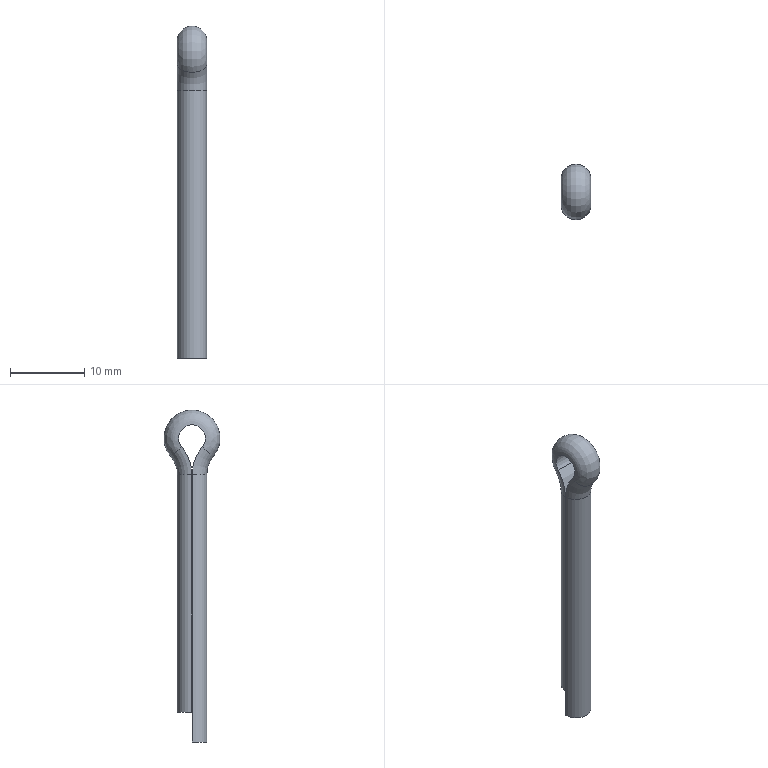Component | NX | 3_COTTER_PIN | 1 solid | 12 faces | box 4 x 7.55 x 44.7 mm | volume 545 mm3 | cylinder 5 | plane 4 | torus 2 | spline 1 | commonest cylinder face diameters 4 x2 11.596 x2 3.596 x1
STEP:
#1=VALUE_REPRESENTATION_ITEM('',COUNT_MEASURE(0.));
#2=(LENGTH_UNIT()NAMED_UNIT(*)SI_UNIT(.MILLI.,.METRE.));
#3=UNCERTAINTY_MEASURE_WITH_UNIT(LENGTH_MEASURE(0.0254),#2,'','');
#4=(NAMED_UNIT(*)PLANE_ANGLE_UNIT()SI_UNIT($,.RADIAN.));
#5=PLANE_ANGLE_MEASURE_WITH_UNIT(PLANE_ANGLE_MEASURE(0.01745),#4);
#6=DIMENSIONAL_EXPONENTS(0.,0.,0.,0.,0.,0.,0.);
#7=(CONVERSION_BASED_UNIT('',#5)NAMED_UNIT(#6)PLANE_ANGLE_UNIT());
#8=(NAMED_UNIT(*)SI_UNIT($,.STERADIAN.)SOLID_ANGLE_UNIT());
#9=(GEOMETRIC_REPRESENTATION_CONTEXT(3)GLOBAL_UNCERTAINTY_ASSIGNED_CONTEXT((#3))GLOBAL_UNIT_ASSIGNED_CONTEXT((#2,#7,#8))REPRESENTATION_CONTEXT('',''));
#10=REPRESENTATION('',(#1),#9);
#11=VALUE_REPRESENTATION_ITEM('',COUNT_MEASURE(0.));
#12=REPRESENTATION('',(#11),#9);
#13=CARTESIAN_POINT('',(0.,0.,0.));
#14=DIRECTION('',(0.,0.,1.));
#15=DIRECTION('',(1.,0.,0.));
#16=AXIS2_PLACEMENT_3D('',#13,#14,#15);
#17=SHAPE_REPRESENTATION('',(#16),#9);
#18=CARTESIAN_POINT('',(36.,-0.005,112.5));
#19=VERTEX_POINT('',#18);
#20=CARTESIAN_POINT('',(40.,-0.005,112.5));
#21=VERTEX_POINT('',#20);
#22=CARTESIAN_POINT('',(36.,-0.005,112.5));
#23=DIRECTION('',(1.,0.,0.));
#24=VECTOR('',#23,1.);
#25=LINE('',#22,#24);
#26=EDGE_CURVE('',#19,#21,#25,.T.);
#27=ORIENTED_EDGE('',*,*,#26,.T.);
#28=CARTESIAN_POINT('',(40.,-0.005,76.5));
#29=VERTEX_POINT('',#28);
#30=CARTESIAN_POINT('',(40.,-0.005,112.5));
#31=DIRECTION('',(0.,0.,-1.));
#32=VECTOR('',#31,1.);
#33=LINE('',#30,#32);
#34=EDGE_CURVE('',#21,#29,#33,.T.);
#35=ORIENTED_EDGE('',*,*,#34,.T.);
#36=CARTESIAN_POINT('',(36.,-0.005,76.5));
#37=VERTEX_POINT('',#36);
#38=CARTESIAN_POINT('',(36.,-0.005,76.5));
#39=DIRECTION('',(1.,0.,0.));
#40=VECTOR('',#39,1.);
#41=LINE('',#38,#40);
#42=EDGE_CURVE('',#37,#29,#41,.T.);
#43=ORIENTED_EDGE('',*,*,#42,.F.);
#44=CARTESIAN_POINT('',(36.,-0.005,112.5));
#45=DIRECTION('',(0.,0.,-1.));
#46=VECTOR('',#45,1.);
#47=LINE('',#44,#46);
#48=EDGE_CURVE('',#19,#37,#47,.T.);
#49=ORIENTED_EDGE('',*,*,#48,.F.);
#50=EDGE_LOOP('',(#27,#35,#43,#49));
#51=FACE_OUTER_BOUND('',#50,.T.);
#52=CARTESIAN_POINT('',(36.,-0.005,112.5));
#53=DIRECTION('',(0.,1.,0.));
#54=DIRECTION('',(0.,0.,1.));
#55=AXIS2_PLACEMENT_3D('',#52,#53,#54);
#56=PLANE('',#55);
#57=ADVANCED_FACE('',(#51),#56,.T.);
#58=CARTESIAN_POINT('',(38.,0.,112.5));
#59=DIRECTION('',(0.,-0.,-1.));
#60=DIRECTION('',(1.,0.,0.));
#61=AXIS2_PLACEMENT_3D('',#58,#59,#60);
#62=CIRCLE('',#61,2.);
#63=EDGE_CURVE('',#21,#19,#62,.T.);
#64=ORIENTED_EDGE('',*,*,#63,.T.);
#65=ORIENTED_EDGE('',*,*,#48,.T.);
#66=CARTESIAN_POINT('',(38.,0.,76.5));
#67=DIRECTION('',(0.,-0.,-1.));
#68=DIRECTION('',(1.,0.,0.));
#69=AXIS2_PLACEMENT_3D('',#66,#67,#68);
#70=CIRCLE('',#69,2.);
#71=EDGE_CURVE('',#29,#37,#70,.T.);
#72=ORIENTED_EDGE('',*,*,#71,.F.);
#73=ORIENTED_EDGE('',*,*,#34,.F.);
#74=EDGE_LOOP('',(#64,#65,#72,#73));
#75=FACE_OUTER_BOUND('',#74,.T.);
#76=CARTESIAN_POINT('',(38.,0.,112.5));
#77=DIRECTION('',(0.,0.,-1.));
#78=DIRECTION('',(-1.,0.,0.));
#79=AXIS2_PLACEMENT_3D('',#76,#77,#78);
#80=CYLINDRICAL_SURFACE('',#79,2.);
#81=ADVANCED_FACE('',(#75),#80,.T.);
#82=CARTESIAN_POINT('',(36.,-1.374,116.241));
#83=VERTEX_POINT('',#82);
#84=CARTESIAN_POINT('',(40.,-1.374,116.241));
#85=VERTEX_POINT('',#84);
#86=CARTESIAN_POINT('',(36.,-1.374,116.241));
#87=DIRECTION('',(1.,0.,0.));
#88=VECTOR('',#87,1.);
#89=LINE('',#86,#88);
#90=EDGE_CURVE('',#83,#85,#89,.T.);
#91=ORIENTED_EDGE('',*,*,#90,.T.);
#92=CARTESIAN_POINT('',(40.,-5.803,112.5));
#93=DIRECTION('',(-1.,0.,0.));
#94=DIRECTION('',(0.,0.,1.));
#95=AXIS2_PLACEMENT_3D('',#92,#93,#94);
#96=CIRCLE('',#95,5.798);
#97=EDGE_CURVE('',#85,#21,#96,.T.);
#98=ORIENTED_EDGE('',*,*,#97,.T.);
#99=ORIENTED_EDGE('',*,*,#26,.F.);
#100=CARTESIAN_POINT('',(36.,-5.803,112.5));
#101=DIRECTION('',(-1.,0.,0.));
#102=DIRECTION('',(0.,0.,1.));
#103=AXIS2_PLACEMENT_3D('',#100,#101,#102);
#104=CIRCLE('',#103,5.798);
#105=EDGE_CURVE('',#83,#19,#104,.T.);
#106=ORIENTED_EDGE('',*,*,#105,.F.);
#107=EDGE_LOOP('',(#91,#98,#99,#106));
#108=FACE_OUTER_BOUND('',#107,.T.);
#109=CARTESIAN_POINT('',(38.,-5.803,112.5));
#110=DIRECTION('',(-1.,0.,0.));
#111=DIRECTION('',(0.,0.,1.));
#112=AXIS2_PLACEMENT_3D('',#109,#110,#111);
#113=CYLINDRICAL_SURFACE('',#112,5.798);
#114=ADVANCED_FACE('',(#108),#113,.T.);
#115=CARTESIAN_POINT('',(38.,-1.37,116.245));
#116=DIRECTION('',(0.,0.6453,-0.7639));
#117=DIRECTION('',(1.,0.,0.));
#118=AXIS2_PLACEMENT_3D('',#115,#116,#117);
#119=CIRCLE('',#118,2.);
#120=EDGE_CURVE('',#85,#83,#119,.T.);
#121=ORIENTED_EDGE('',*,*,#120,.T.);
#122=ORIENTED_EDGE('',*,*,#105,.T.);
#123=ORIENTED_EDGE('',*,*,#63,.F.);
#124=ORIENTED_EDGE('',*,*,#97,.F.);
#125=EDGE_LOOP('',(#121,#122,#123,#124));
#126=FACE_OUTER_BOUND('',#125,.T.);
#127=CARTESIAN_POINT('',(38.,-5.803,112.5));
#128=DIRECTION('',(-1.,0.,0.));
#129=DIRECTION('',(0.,0.,1.));
#130=AXIS2_PLACEMENT_3D('',#127,#128,#129);
#131=TOROIDAL_SURFACE('',#130,5.803,2.);
#132=ADVANCED_FACE('',(#126),#131,.T.);
#133=CARTESIAN_POINT('',(36.,1.374,116.241));
#134=VERTEX_POINT('',#133);
#135=CARTESIAN_POINT('',(40.,1.374,116.241));
#136=VERTEX_POINT('',#135);
#137=CARTESIAN_POINT('',(36.,1.374,116.241));
#138=DIRECTION('',(1.,0.,0.));
#139=VECTOR('',#138,1.);
#140=LINE('',#137,#139);
#141=EDGE_CURVE('',#134,#136,#140,.T.);
#142=ORIENTED_EDGE('',*,*,#141,.T.);
#143=CARTESIAN_POINT('',(40.,0.,117.402));
#144=DIRECTION('',(1.,0.,0.));
#145=DIRECTION('',(0.,0.,-1.));
#146=AXIS2_PLACEMENT_3D('',#143,#144,#145);
#147=CIRCLE('',#146,1.798);
#148=EDGE_CURVE('',#136,#85,#147,.T.);
#149=ORIENTED_EDGE('',*,*,#148,.T.);
#150=ORIENTED_EDGE('',*,*,#90,.F.);
#151=CARTESIAN_POINT('',(36.,0.,117.402));
#152=DIRECTION('',(1.,0.,0.));
#153=DIRECTION('',(0.,0.,-1.));
#154=AXIS2_PLACEMENT_3D('',#151,#152,#153);
#155=CIRCLE('',#154,1.798);
#156=EDGE_CURVE('',#134,#83,#155,.T.);
#157=ORIENTED_EDGE('',*,*,#156,.F.);
#158=EDGE_LOOP('',(#142,#149,#150,#157));
#159=FACE_OUTER_BOUND('',#158,.T.);
#160=CARTESIAN_POINT('',(38.,0.,117.402));
#161=DIRECTION('',(1.,0.,0.));
#162=DIRECTION('',(0.,0.,-1.));
#163=AXIS2_PLACEMENT_3D('',#160,#161,#162);
#164=CYLINDRICAL_SURFACE('',#163,1.798);
#165=ADVANCED_FACE('',(#159),#164,.F.);
#166=CARTESIAN_POINT('',(38.,1.37,116.245));
#167=DIRECTION('',(0.,0.6453,0.7639));
#168=DIRECTION('',(1.,0.,0.));
#169=AXIS2_PLACEMENT_3D('',#166,#167,#168);
#170=CIRCLE('',#169,2.);
#171=EDGE_CURVE('',#136,#134,#170,.T.);
#172=ORIENTED_EDGE('',*,*,#171,.T.);
#173=ORIENTED_EDGE('',*,*,#156,.T.);
#174=ORIENTED_EDGE('',*,*,#120,.F.);
#175=ORIENTED_EDGE('',*,*,#148,.F.);
#176=EDGE_LOOP('',(#172,#173,#174,#175));
#177=FACE_OUTER_BOUND('',#176,.T.);
#178=CARTESIAN_POINT('',(40.,1.374,116.241));
#179=CARTESIAN_POINT('',(40.,2.516,117.594));
#180=CARTESIAN_POINT('',(40.,1.771,119.2));
#181=CARTESIAN_POINT('',(40.,0.,119.2));
#182=CARTESIAN_POINT('',(40.,-1.771,119.2));
#183=CARTESIAN_POINT('',(40.,-2.516,117.594));
#184=CARTESIAN_POINT('',(40.,-1.374,116.241));
#185=CARTESIAN_POINT('',(39.99,4.414,113.673));
#186=CARTESIAN_POINT('',(39.99,8.086,118.02));
#187=CARTESIAN_POINT('',(39.99,5.69,123.18));
#188=CARTESIAN_POINT('',(39.99,0.,123.18));
#189=CARTESIAN_POINT('',(39.99,-5.69,123.18));
#190=CARTESIAN_POINT('',(39.99,-8.086,118.02));
#191=CARTESIAN_POINT('',(39.99,-4.414,113.673));
#192=CARTESIAN_POINT('',(36.01,4.414,113.673));
#193=CARTESIAN_POINT('',(36.01,8.086,118.02));
#194=CARTESIAN_POINT('',(36.01,5.69,123.18));
#195=CARTESIAN_POINT('',(36.01,0.,123.18));
#196=CARTESIAN_POINT('',(36.01,-5.69,123.18));
#197=CARTESIAN_POINT('',(36.01,-8.086,118.02));
#198=CARTESIAN_POINT('',(36.01,-4.414,113.673));
#199=CARTESIAN_POINT('',(36.,1.374,116.241));
#200=CARTESIAN_POINT('',(36.,2.516,117.594));
#201=CARTESIAN_POINT('',(36.,1.771,119.2));
#202=CARTESIAN_POINT('',(36.,0.,119.2));
#203=CARTESIAN_POINT('',(36.,-1.771,119.2));
#204=CARTESIAN_POINT('',(36.,-2.516,117.594));
#205=CARTESIAN_POINT('',(36.,-1.374,116.241));
#206=(BOUNDED_SURFACE()B_SPLINE_SURFACE(3,3,((#178,#179,#180,#181,#182,#183,#184),(#185,#186,#187,#188,#189,#190,#191),(#192,#193,#194,#195,#196,#197,#198),(#199,#200,#201,#202,#203,#204,#205)),.UNSPECIFIED.,.F.,.F.,.F.)B_SPLINE_SURFACE_WITH_KNOTS((4,4),(4,3,4),(0.,1.),(0.,0.5,1.),.UNSPECIFIED.)GEOMETRIC_REPRESENTATION_ITEM()RATIONAL_B_SPLINE_SURFACE(((1.,0.6141,0.6141,1.,0.6141,0.6141,1.),(0.335,0.2057,0.2057,0.335,0.2057,0.2057,0.335),(0.335,0.2057,0.2057,0.335,0.2057,0.2057,0.335),(1.,0.6141,0.6141,1.,0.6141,0.6141,1.)))REPRESENTATION_ITEM('')SURFACE());
#207=ADVANCED_FACE('',(#177),#206,.T.);
#208=CARTESIAN_POINT('',(36.,0.005,112.5));
#209=VERTEX_POINT('',#208);
#210=CARTESIAN_POINT('',(40.,0.005,112.5));
#211=VERTEX_POINT('',#210);
#212=CARTESIAN_POINT('',(36.,0.005,112.5));
#213=DIRECTION('',(1.,0.,0.));
#214=VECTOR('',#213,1.);
#215=LINE('',#212,#214);
#216=EDGE_CURVE('',#209,#211,#215,.T.);
#217=ORIENTED_EDGE('',*,*,#216,.T.);
#218=CARTESIAN_POINT('',(40.,5.803,112.5));
#219=DIRECTION('',(-1.,0.,0.));
#220=DIRECTION('',(0.,0.,1.));
#221=AXIS2_PLACEMENT_3D('',#218,#219,#220);
#222=CIRCLE('',#221,5.798);
#223=EDGE_CURVE('',#211,#136,#222,.T.);
#224=ORIENTED_EDGE('',*,*,#223,.T.);
#225=ORIENTED_EDGE('',*,*,#141,.F.);
#226=CARTESIAN_POINT('',(36.,5.803,112.5));
#227=DIRECTION('',(-1.,0.,0.));
#228=DIRECTION('',(0.,0.,1.));
#229=AXIS2_PLACEMENT_3D('',#226,#227,#228);
#230=CIRCLE('',#229,5.798);
#231=EDGE_CURVE('',#209,#134,#230,.T.);
#232=ORIENTED_EDGE('',*,*,#231,.F.);
#233=EDGE_LOOP('',(#217,#224,#225,#232));
#234=FACE_OUTER_BOUND('',#233,.T.);
#235=CARTESIAN_POINT('',(38.,5.803,112.5));
#236=DIRECTION('',(-1.,0.,0.));
#237=DIRECTION('',(0.,0.,1.));
#238=AXIS2_PLACEMENT_3D('',#235,#236,#237);
#239=CYLINDRICAL_SURFACE('',#238,5.798);
#240=ADVANCED_FACE('',(#234),#239,.T.);
#241=CARTESIAN_POINT('',(38.,0.,112.5));
#242=DIRECTION('',(0.,0.,1.));
#243=DIRECTION('',(1.,0.,0.));
#244=AXIS2_PLACEMENT_3D('',#241,#242,#243);
#245=CIRCLE('',#244,2.);
#246=EDGE_CURVE('',#211,#209,#245,.T.);
#247=ORIENTED_EDGE('',*,*,#246,.T.);
#248=ORIENTED_EDGE('',*,*,#231,.T.);
#249=ORIENTED_EDGE('',*,*,#171,.F.);
#250=ORIENTED_EDGE('',*,*,#223,.F.);
#251=EDGE_LOOP('',(#247,#248,#249,#250));
#252=FACE_OUTER_BOUND('',#251,.T.);
#253=CARTESIAN_POINT('',(38.,5.803,112.5));
#254=DIRECTION('',(-1.,0.,0.));
#255=DIRECTION('',(0.,0.,1.));
#256=AXIS2_PLACEMENT_3D('',#253,#254,#255);
#257=TOROIDAL_SURFACE('',#256,5.803,2.);
#258=ADVANCED_FACE('',(#252),#257,.T.);
#259=CARTESIAN_POINT('',(40.,0.005,80.5));
#260=VERTEX_POINT('',#259);
#261=CARTESIAN_POINT('',(36.,0.005,80.5));
#262=VERTEX_POINT('',#261);
#263=CARTESIAN_POINT('',(38.,0.,80.5));
#264=DIRECTION('',(0.,0.,1.));
#265=DIRECTION('',(1.,0.,0.));
#266=AXIS2_PLACEMENT_3D('',#263,#264,#265);
#267=CIRCLE('',#266,2.);
#268=EDGE_CURVE('',#260,#262,#267,.T.);
#269=ORIENTED_EDGE('',*,*,#268,.T.);
#270=CARTESIAN_POINT('',(36.,0.005,112.5));
#271=DIRECTION('',(0.,0.,-1.));
#272=VECTOR('',#271,1.);
#273=LINE('',#270,#272);
#274=EDGE_CURVE('',#209,#262,#273,.T.);
#275=ORIENTED_EDGE('',*,*,#274,.F.);
#276=ORIENTED_EDGE('',*,*,#246,.F.);
#277=CARTESIAN_POINT('',(40.,0.005,112.5));
#278=DIRECTION('',(0.,0.,-1.));
#279=VECTOR('',#278,1.);
#280=LINE('',#277,#279);
#281=EDGE_CURVE('',#211,#260,#280,.T.);
#282=ORIENTED_EDGE('',*,*,#281,.T.);
#283=EDGE_LOOP('',(#269,#275,#276,#282));
#284=FACE_OUTER_BOUND('',#283,.T.);
#285=CARTESIAN_POINT('',(38.,0.,112.5));
#286=DIRECTION('',(0.,0.,-1.));
#287=DIRECTION('',(-1.,0.,0.));
#288=AXIS2_PLACEMENT_3D('',#285,#286,#287);
#289=CYLINDRICAL_SURFACE('',#288,2.);
#290=ADVANCED_FACE('',(#284),#289,.T.);
#291=CARTESIAN_POINT('',(36.,0.005,80.5));
#292=DIRECTION('',(1.,0.,0.));
#293=VECTOR('',#292,1.);
#294=LINE('',#291,#293);
#295=EDGE_CURVE('',#262,#260,#294,.T.);
#296=ORIENTED_EDGE('',*,*,#295,.T.);
#297=ORIENTED_EDGE('',*,*,#281,.F.);
#298=ORIENTED_EDGE('',*,*,#216,.F.);
#299=ORIENTED_EDGE('',*,*,#274,.T.);
#300=EDGE_LOOP('',(#296,#297,#298,#299));
#301=FACE_OUTER_BOUND('',#300,.T.);
#302=CARTESIAN_POINT('',(36.,0.005,112.5));
#303=DIRECTION('',(0.,1.,0.));
#304=DIRECTION('',(0.,0.,1.));
#305=AXIS2_PLACEMENT_3D('',#302,#303,#304);
#306=PLANE('',#305);
#307=ADVANCED_FACE('',(#301),#306,.F.);
#308=ORIENTED_EDGE('',*,*,#71,.T.);
#309=ORIENTED_EDGE('',*,*,#42,.T.);
#310=EDGE_LOOP('',(#308,#309));
#311=FACE_OUTER_BOUND('',#310,.T.);
#312=CARTESIAN_POINT('',(38.,0.,76.5));
#313=DIRECTION('',(0.,-0.,-1.));
#314=DIRECTION('',(1.,0.,0.));
#315=AXIS2_PLACEMENT_3D('',#312,#313,#314);
#316=PLANE('',#315);
#317=ADVANCED_FACE('',(#311),#316,.T.);
#318=ORIENTED_EDGE('',*,*,#268,.F.);
#319=ORIENTED_EDGE('',*,*,#295,.F.);
#320=EDGE_LOOP('',(#318,#319));
#321=FACE_OUTER_BOUND('',#320,.T.);
#322=CARTESIAN_POINT('',(38.,0.,80.5));
#323=DIRECTION('',(0.,0.,1.));
#324=DIRECTION('',(1.,0.,0.));
#325=AXIS2_PLACEMENT_3D('',#322,#323,#324);
#326=PLANE('',#325);
#327=ADVANCED_FACE('',(#321),#326,.F.);
#328=CLOSED_SHELL('',(#57,#81,#114,#132,#165,#207,#240,#258,#290,#307,#317,#327));
#329=MANIFOLD_SOLID_BREP('',#328);
#330=ADVANCED_BREP_SHAPE_REPRESENTATION('',(#329),#9);
#331=SHAPE_REPRESENTATION_RELATIONSHIP('','',#17,#330);
#332=PRESENTATION_LAYER_ASSIGNMENT('','',(#329));
#333=COLOUR_RGB('',0.6,0.6,0.6);
#334=FILL_AREA_STYLE_COLOUR('',#333);
#335=FILL_AREA_STYLE('',(#334));
#336=SURFACE_STYLE_FILL_AREA(#335);
#337=SURFACE_SIDE_STYLE('',(#336));
#338=SURFACE_STYLE_USAGE(.BOTH.,#337);
#339=PRESENTATION_STYLE_ASSIGNMENT((#338));
#340=STYLED_ITEM('',(#339),#329);
#341=MECHANICAL_DESIGN_GEOMETRIC_PRESENTATION_REPRESENTATION('',(#340),#9);